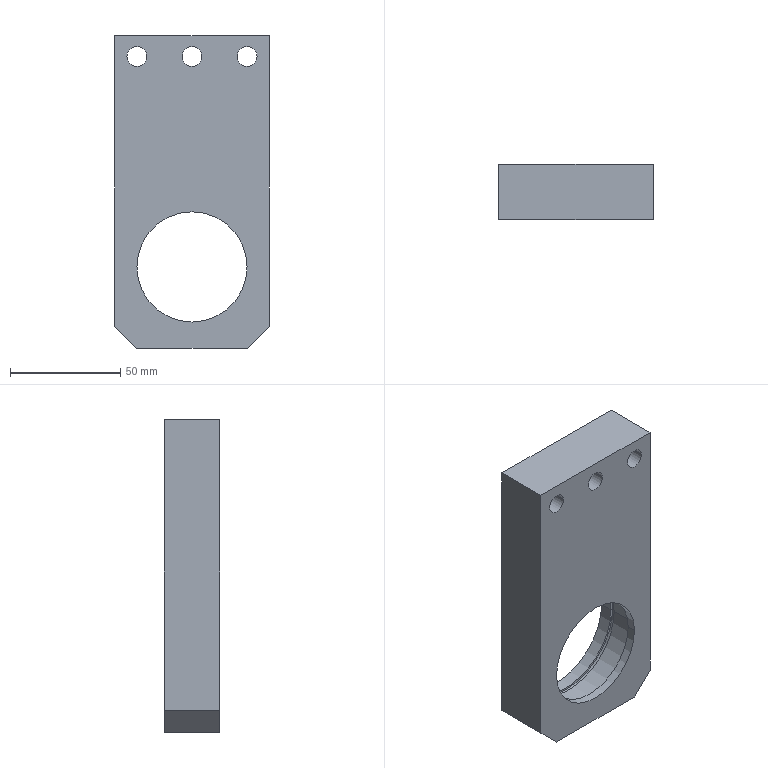Component | SolidWorks | -SlidingBearingHousing-1 | 1 solid | 34 faces | box 70 x 25 x 142 mm | volume 175353 mm3 | cylinder 20 | plane 14 | commonest cylinder face diameters 14 x6 9 x6 58 x4 60 x2 50 x2
build123d program:
from build123d import *

# Parameters (mm, degrees)
BOSS_EXTRUDE1_DEPTH = 25
SKETCH9_R           = 4.5
CUT_EXTRUDE5_DEPTH  = 84.012
SKETCH11_R          = 7
CUT_EXTRUDE6_DEPTH  = 8


with BuildPart() as part:
    # Sketch1 → Boss-Extrude1 (new body)
    with BuildSketch(Plane.XY):
        Polygon((-35, 61), (-25, 71), (25, 71), (35, 61), (35, -71), (-35, -71), align=None)
    extrude(amount=BOSS_EXTRUDE1_DEPTH)

    # Sketch9 → Cut-Extrude5 (cut, through all)
    with BuildSketch(Plane(origin=(0, 0, 0), x_dir=(-1, 0, 0), z_dir=(0, 0, -1))):
        with Locations((-25, -61.5)):
            Circle(SKETCH9_R)
        with Locations((0, -61.5)):
            Circle(SKETCH9_R)
        with Locations((25, -61.5)):
            Circle(SKETCH9_R)
    extrude(amount=-CUT_EXTRUDE5_DEPTH, mode=Mode.SUBTRACT)

    # Sketch10 → Cut-Revolve1 (revolve, cut)
    with BuildSketch(Plane(origin=(0, 0, 0), x_dir=(0, 0, -1), z_dir=(1, 0, 0)), mode=Mode.PRIVATE) as cut_revolve1_sk:
        Polygon((-25, 59), (-21, 59), (-21, 63), (-8, 63), (-8, 64), (-6, 64), (-6, 63), (0, 63), (0, 34), (-25, 34), align=None)
    revolve(cut_revolve1_sk.sketch.rotate(Axis((0, 34, 57.258), (0, 0, -1)), 90), axis=Axis((0, 34, 57.258), (0, 0, -1)), mode=Mode.SUBTRACT)

    # Sketch11 → Cut-Extrude6 (cut)
    with BuildSketch(Plane(origin=(0, 0, 0), x_dir=(-1, 0, 0), z_dir=(0, 0, -1))):
        with Locations((0, -61.5)):
            Circle(SKETCH11_R)
        with Locations((-25, -61.5)):
            Circle(SKETCH11_R)
        with Locations((25, -61.5)):
            Circle(SKETCH11_R)
    extrude(amount=-CUT_EXTRUDE6_DEPTH, mode=Mode.SUBTRACT)


solid = part.part

# Placed as in the assembly
solid = solid.moved(Location((205, 1334.5, -139), (90, 0, -180)))
STEP:
#1=COLOUR_RGB('',0.7922,0.8196,0.9333);
#2=FILL_AREA_STYLE_COLOUR('',#1);
#3=FILL_AREA_STYLE('',(#2));
#4=SURFACE_STYLE_FILL_AREA(#3);
#5=SURFACE_SIDE_STYLE('',(#4));
#6=SURFACE_STYLE_USAGE(.BOTH.,#5);
#7=PRESENTATION_STYLE_ASSIGNMENT((#6));
#8=CARTESIAN_POINT('',(8.78,52.224,-3.051));
#9=VERTEX_POINT('',#8);
#10=CARTESIAN_POINT('',(9.331,52.224,-3.051));
#11=VERTEX_POINT('',#10);
#12=CARTESIAN_POINT('',(9.055,52.224,-3.051));
#13=DIRECTION('',(-0.,1.,-0.));
#14=DIRECTION('',(1.,0.,0.));
#15=AXIS2_PLACEMENT_3D('',#12,#13,#14);
#16=CIRCLE('',#15,0.2756);
#17=EDGE_CURVE('',#9,#11,#16,.T.);
#18=ORIENTED_EDGE('',*,*,#17,.F.);
#19=CARTESIAN_POINT('',(8.78,52.539,-3.051));
#20=VERTEX_POINT('',#19);
#21=CARTESIAN_POINT('',(8.78,52.224,-3.051));
#22=DIRECTION('',(-0.,1.,-0.));
#23=VECTOR('',#22,39.37);
#24=LINE('',#21,#23);
#25=EDGE_CURVE('',#9,#20,#24,.T.);
#26=ORIENTED_EDGE('',*,*,#25,.T.);
#27=CARTESIAN_POINT('',(9.331,52.539,-3.051));
#28=VERTEX_POINT('',#27);
#29=CARTESIAN_POINT('',(9.055,52.539,-3.051));
#30=DIRECTION('',(-0.,1.,-0.));
#31=DIRECTION('',(1.,0.,0.));
#32=AXIS2_PLACEMENT_3D('',#29,#30,#31);
#33=CIRCLE('',#32,0.2756);
#34=EDGE_CURVE('',#20,#28,#33,.T.);
#35=ORIENTED_EDGE('',*,*,#34,.T.);
#36=CARTESIAN_POINT('',(9.331,52.224,-3.051));
#37=DIRECTION('',(-0.,1.,-0.));
#38=VECTOR('',#37,39.37);
#39=LINE('',#36,#38);
#40=EDGE_CURVE('',#11,#28,#39,.T.);
#41=ORIENTED_EDGE('',*,*,#40,.F.);
#42=EDGE_LOOP('',(#18,#26,#35,#41));
#43=FACE_OUTER_BOUND('',#42,.T.);
#44=CARTESIAN_POINT('',(9.055,52.224,-3.051));
#45=DIRECTION('',(-0.,1.,-0.));
#46=DIRECTION('',(1.,0.,0.));
#47=AXIS2_PLACEMENT_3D('',#44,#45,#46);
#48=CYLINDRICAL_SURFACE('',#47,0.2756);
#49=ADVANCED_FACE('',(#43),#48,.F.);
#50=CARTESIAN_POINT('',(6.811,52.224,-3.051));
#51=VERTEX_POINT('',#50);
#52=CARTESIAN_POINT('',(7.362,52.224,-3.051));
#53=VERTEX_POINT('',#52);
#54=CARTESIAN_POINT('',(7.087,52.224,-3.051));
#55=DIRECTION('',(-0.,1.,-0.));
#56=DIRECTION('',(1.,0.,0.));
#57=AXIS2_PLACEMENT_3D('',#54,#55,#56);
#58=CIRCLE('',#57,0.2756);
#59=EDGE_CURVE('',#51,#53,#58,.T.);
#60=ORIENTED_EDGE('',*,*,#59,.F.);
#61=CARTESIAN_POINT('',(6.811,52.539,-3.051));
#62=VERTEX_POINT('',#61);
#63=CARTESIAN_POINT('',(6.811,52.224,-3.051));
#64=DIRECTION('',(-0.,1.,-0.));
#65=VECTOR('',#64,39.37);
#66=LINE('',#63,#65);
#67=EDGE_CURVE('',#51,#62,#66,.T.);
#68=ORIENTED_EDGE('',*,*,#67,.T.);
#69=CARTESIAN_POINT('',(7.362,52.539,-3.051));
#70=VERTEX_POINT('',#69);
#71=CARTESIAN_POINT('',(7.087,52.539,-3.051));
#72=DIRECTION('',(-0.,1.,-0.));
#73=DIRECTION('',(1.,0.,0.));
#74=AXIS2_PLACEMENT_3D('',#71,#72,#73);
#75=CIRCLE('',#74,0.2756);
#76=EDGE_CURVE('',#62,#70,#75,.T.);
#77=ORIENTED_EDGE('',*,*,#76,.T.);
#78=CARTESIAN_POINT('',(7.362,52.224,-3.051));
#79=DIRECTION('',(-0.,1.,-0.));
#80=VECTOR('',#79,39.37);
#81=LINE('',#78,#80);
#82=EDGE_CURVE('',#53,#70,#81,.T.);
#83=ORIENTED_EDGE('',*,*,#82,.F.);
#84=EDGE_LOOP('',(#60,#68,#77,#83));
#85=FACE_OUTER_BOUND('',#84,.T.);
#86=CARTESIAN_POINT('',(7.087,52.224,-3.051));
#87=DIRECTION('',(-0.,1.,-0.));
#88=DIRECTION('',(1.,0.,0.));
#89=AXIS2_PLACEMENT_3D('',#86,#87,#88);
#90=CYLINDRICAL_SURFACE('',#89,0.2756);
#91=ADVANCED_FACE('',(#85),#90,.F.);
#92=CARTESIAN_POINT('',(7.795,52.224,-3.051));
#93=VERTEX_POINT('',#92);
#94=CARTESIAN_POINT('',(8.346,52.224,-3.051));
#95=VERTEX_POINT('',#94);
#96=CARTESIAN_POINT('',(8.071,52.224,-3.051));
#97=DIRECTION('',(-0.,1.,-0.));
#98=DIRECTION('',(1.,0.,0.));
#99=AXIS2_PLACEMENT_3D('',#96,#97,#98);
#100=CIRCLE('',#99,0.2756);
#101=EDGE_CURVE('',#93,#95,#100,.T.);
#102=ORIENTED_EDGE('',*,*,#101,.F.);
#103=CARTESIAN_POINT('',(7.795,52.539,-3.051));
#104=VERTEX_POINT('',#103);
#105=CARTESIAN_POINT('',(7.795,52.224,-3.051));
#106=DIRECTION('',(-0.,1.,-0.));
#107=VECTOR('',#106,39.37);
#108=LINE('',#105,#107);
#109=EDGE_CURVE('',#93,#104,#108,.T.);
#110=ORIENTED_EDGE('',*,*,#109,.T.);
#111=CARTESIAN_POINT('',(8.346,52.539,-3.051));
#112=VERTEX_POINT('',#111);
#113=CARTESIAN_POINT('',(8.071,52.539,-3.051));
#114=DIRECTION('',(-0.,1.,-0.));
#115=DIRECTION('',(1.,0.,0.));
#116=AXIS2_PLACEMENT_3D('',#113,#114,#115);
#117=CIRCLE('',#116,0.2756);
#118=EDGE_CURVE('',#104,#112,#117,.T.);
#119=ORIENTED_EDGE('',*,*,#118,.T.);
#120=CARTESIAN_POINT('',(8.346,52.224,-3.051));
#121=DIRECTION('',(-0.,1.,-0.));
#122=VECTOR('',#121,39.37);
#123=LINE('',#120,#122);
#124=EDGE_CURVE('',#95,#112,#123,.T.);
#125=ORIENTED_EDGE('',*,*,#124,.F.);
#126=EDGE_LOOP('',(#102,#110,#119,#125));
#127=FACE_OUTER_BOUND('',#126,.T.);
#128=CARTESIAN_POINT('',(8.071,52.224,-3.051));
#129=DIRECTION('',(-0.,1.,-0.));
#130=DIRECTION('',(1.,0.,0.));
#131=AXIS2_PLACEMENT_3D('',#128,#129,#130);
#132=CYLINDRICAL_SURFACE('',#131,0.2756);
#133=ADVANCED_FACE('',(#127),#132,.F.);
#134=CARTESIAN_POINT('',(9.213,52.539,-6.811));
#135=VERTEX_POINT('',#134);
#136=CARTESIAN_POINT('',(6.929,52.539,-6.811));
#137=VERTEX_POINT('',#136);
#138=CARTESIAN_POINT('',(8.071,52.539,-6.811));
#139=DIRECTION('',(0.,-1.,0.));
#140=DIRECTION('',(-1.,0.,0.));
#141=AXIS2_PLACEMENT_3D('',#138,#139,#140);
#142=CIRCLE('',#141,1.142);
#143=EDGE_CURVE('',#135,#137,#142,.T.);
#144=ORIENTED_EDGE('',*,*,#143,.F.);
#145=CARTESIAN_POINT('',(9.213,52.303,-6.811));
#146=VERTEX_POINT('',#145);
#147=CARTESIAN_POINT('',(9.213,50.285,-6.811));
#148=DIRECTION('',(0.,-1.,0.));
#149=VECTOR('',#148,39.37);
#150=LINE('',#147,#149);
#151=EDGE_CURVE('',#135,#146,#150,.T.);
#152=ORIENTED_EDGE('',*,*,#151,.T.);
#153=CARTESIAN_POINT('',(6.929,52.303,-6.811));
#154=VERTEX_POINT('',#153);
#155=CARTESIAN_POINT('',(8.071,52.303,-6.811));
#156=DIRECTION('',(0.,-1.,0.));
#157=DIRECTION('',(-1.,0.,0.));
#158=AXIS2_PLACEMENT_3D('',#155,#156,#157);
#159=CIRCLE('',#158,1.142);
#160=EDGE_CURVE('',#146,#154,#159,.T.);
#161=ORIENTED_EDGE('',*,*,#160,.T.);
#162=CARTESIAN_POINT('',(6.929,50.285,-6.811));
#163=DIRECTION('',(0.,-1.,0.));
#164=VECTOR('',#163,39.37);
#165=LINE('',#162,#164);
#166=EDGE_CURVE('',#137,#154,#165,.T.);
#167=ORIENTED_EDGE('',*,*,#166,.F.);
#168=EDGE_LOOP('',(#144,#152,#161,#167));
#169=FACE_OUTER_BOUND('',#168,.T.);
#170=CARTESIAN_POINT('',(8.071,50.285,-6.811));
#171=DIRECTION('',(0.,-1.,0.));
#172=DIRECTION('',(-1.,0.,0.));
#173=AXIS2_PLACEMENT_3D('',#170,#171,#172);
#174=CYLINDRICAL_SURFACE('',#173,1.142);
#175=ADVANCED_FACE('',(#169),#174,.F.);
#176=CARTESIAN_POINT('',(9.252,52.303,-6.811));
#177=VERTEX_POINT('',#176);
#178=CARTESIAN_POINT('',(6.89,52.303,-6.811));
#179=VERTEX_POINT('',#178);
#180=CARTESIAN_POINT('',(8.071,52.303,-6.811));
#181=DIRECTION('',(0.,-1.,0.));
#182=DIRECTION('',(-1.,0.,0.));
#183=AXIS2_PLACEMENT_3D('',#180,#181,#182);
#184=CIRCLE('',#183,1.181);
#185=EDGE_CURVE('',#177,#179,#184,.T.);
#186=ORIENTED_EDGE('',*,*,#185,.F.);
#187=CARTESIAN_POINT('',(9.252,52.224,-6.811));
#188=VERTEX_POINT('',#187);
#189=CARTESIAN_POINT('',(9.252,50.285,-6.811));
#190=DIRECTION('',(0.,-1.,0.));
#191=VECTOR('',#190,39.37);
#192=LINE('',#189,#191);
#193=EDGE_CURVE('',#177,#188,#192,.T.);
#194=ORIENTED_EDGE('',*,*,#193,.T.);
#195=CARTESIAN_POINT('',(6.89,52.224,-6.811));
#196=VERTEX_POINT('',#195);
#197=CARTESIAN_POINT('',(8.071,52.224,-6.811));
#198=DIRECTION('',(0.,-1.,0.));
#199=DIRECTION('',(-1.,0.,0.));
#200=AXIS2_PLACEMENT_3D('',#197,#198,#199);
#201=CIRCLE('',#200,1.181);
#202=EDGE_CURVE('',#188,#196,#201,.T.);
#203=ORIENTED_EDGE('',*,*,#202,.T.);
#204=CARTESIAN_POINT('',(6.89,50.285,-6.811));
#205=DIRECTION('',(0.,-1.,0.));
#206=VECTOR('',#205,39.37);
#207=LINE('',#204,#206);
#208=EDGE_CURVE('',#179,#196,#207,.T.);
#209=ORIENTED_EDGE('',*,*,#208,.F.);
#210=EDGE_LOOP('',(#186,#194,#203,#209));
#211=FACE_OUTER_BOUND('',#210,.T.);
#212=CARTESIAN_POINT('',(8.071,50.285,-6.811));
#213=DIRECTION('',(0.,-1.,0.));
#214=DIRECTION('',(-1.,0.,0.));
#215=AXIS2_PLACEMENT_3D('',#212,#213,#214);
#216=CYLINDRICAL_SURFACE('',#215,1.181);
#217=ADVANCED_FACE('',(#211),#216,.F.);
#218=CARTESIAN_POINT('',(9.213,52.224,-6.811));
#219=VERTEX_POINT('',#218);
#220=CARTESIAN_POINT('',(6.929,52.224,-6.811));
#221=VERTEX_POINT('',#220);
#222=CARTESIAN_POINT('',(8.071,52.224,-6.811));
#223=DIRECTION('',(0.,-1.,0.));
#224=DIRECTION('',(-1.,0.,0.));
#225=AXIS2_PLACEMENT_3D('',#222,#223,#224);
#226=CIRCLE('',#225,1.142);
#227=EDGE_CURVE('',#219,#221,#226,.T.);
#228=ORIENTED_EDGE('',*,*,#227,.F.);
#229=CARTESIAN_POINT('',(9.213,51.713,-6.811));
#230=VERTEX_POINT('',#229);
#231=CARTESIAN_POINT('',(9.213,50.285,-6.811));
#232=DIRECTION('',(0.,-1.,0.));
#233=VECTOR('',#232,39.37);
#234=LINE('',#231,#233);
#235=EDGE_CURVE('',#219,#230,#234,.T.);
#236=ORIENTED_EDGE('',*,*,#235,.T.);
#237=CARTESIAN_POINT('',(6.929,51.713,-6.811));
#238=VERTEX_POINT('',#237);
#239=CARTESIAN_POINT('',(8.071,51.713,-6.811));
#240=DIRECTION('',(0.,-1.,0.));
#241=DIRECTION('',(-1.,0.,0.));
#242=AXIS2_PLACEMENT_3D('',#239,#240,#241);
#243=CIRCLE('',#242,1.142);
#244=EDGE_CURVE('',#230,#238,#243,.T.);
#245=ORIENTED_EDGE('',*,*,#244,.T.);
#246=CARTESIAN_POINT('',(6.929,50.285,-6.811));
#247=DIRECTION('',(0.,-1.,0.));
#248=VECTOR('',#247,39.37);
#249=LINE('',#246,#248);
#250=EDGE_CURVE('',#221,#238,#249,.T.);
#251=ORIENTED_EDGE('',*,*,#250,.F.);
#252=EDGE_LOOP('',(#228,#236,#245,#251));
#253=FACE_OUTER_BOUND('',#252,.T.);
#254=CARTESIAN_POINT('',(8.071,50.285,-6.811));
#255=DIRECTION('',(0.,-1.,0.));
#256=DIRECTION('',(-1.,0.,0.));
#257=AXIS2_PLACEMENT_3D('',#254,#255,#256);
#258=CYLINDRICAL_SURFACE('',#257,1.142);
#259=ADVANCED_FACE('',(#253),#258,.F.);
#260=CARTESIAN_POINT('',(9.055,51.713,-6.811));
#261=VERTEX_POINT('',#260);
#262=CARTESIAN_POINT('',(7.087,51.713,-6.811));
#263=VERTEX_POINT('',#262);
#264=CARTESIAN_POINT('',(8.071,51.713,-6.811));
#265=DIRECTION('',(0.,-1.,0.));
#266=DIRECTION('',(-1.,0.,0.));
#267=AXIS2_PLACEMENT_3D('',#264,#265,#266);
#268=CIRCLE('',#267,0.9843);
#269=EDGE_CURVE('',#261,#263,#268,.T.);
#270=ORIENTED_EDGE('',*,*,#269,.F.);
#271=CARTESIAN_POINT('',(9.055,51.555,-6.811));
#272=VERTEX_POINT('',#271);
#273=CARTESIAN_POINT('',(9.055,50.285,-6.811));
#274=DIRECTION('',(0.,-1.,0.));
#275=VECTOR('',#274,39.37);
#276=LINE('',#273,#275);
#277=EDGE_CURVE('',#261,#272,#276,.T.);
#278=ORIENTED_EDGE('',*,*,#277,.T.);
#279=CARTESIAN_POINT('',(7.087,51.555,-6.811));
#280=VERTEX_POINT('',#279);
#281=CARTESIAN_POINT('',(8.071,51.555,-6.811));
#282=DIRECTION('',(0.,-1.,0.));
#283=DIRECTION('',(-1.,0.,0.));
#284=AXIS2_PLACEMENT_3D('',#281,#282,#283);
#285=CIRCLE('',#284,0.9843);
#286=EDGE_CURVE('',#272,#280,#285,.T.);
#287=ORIENTED_EDGE('',*,*,#286,.T.);
#288=CARTESIAN_POINT('',(7.087,50.285,-6.811));
#289=DIRECTION('',(0.,-1.,0.));
#290=VECTOR('',#289,39.37);
#291=LINE('',#288,#290);
#292=EDGE_CURVE('',#263,#280,#291,.T.);
#293=ORIENTED_EDGE('',*,*,#292,.F.);
#294=EDGE_LOOP('',(#270,#278,#287,#293));
#295=FACE_OUTER_BOUND('',#294,.T.);
#296=CARTESIAN_POINT('',(8.071,50.285,-6.811));
#297=DIRECTION('',(0.,-1.,0.));
#298=DIRECTION('',(-1.,0.,0.));
#299=AXIS2_PLACEMENT_3D('',#296,#297,#298);
#300=CYLINDRICAL_SURFACE('',#299,0.9843);
#301=ADVANCED_FACE('',(#295),#300,.F.);
#302=CARTESIAN_POINT('',(7.894,51.555,-3.051));
#303=VERTEX_POINT('',#302);
#304=CARTESIAN_POINT('',(8.248,51.555,-3.051));
#305=VERTEX_POINT('',#304);
#306=CARTESIAN_POINT('',(8.071,51.555,-3.051));
#307=DIRECTION('',(-0.,1.,-0.));
#308=DIRECTION('',(1.,0.,0.));
#309=AXIS2_PLACEMENT_3D('',#306,#307,#308);
#310=CIRCLE('',#309,0.1772);
#311=EDGE_CURVE('',#303,#305,#310,.T.);
#312=ORIENTED_EDGE('',*,*,#311,.F.);
#313=CARTESIAN_POINT('',(7.894,52.224,-3.051));
#314=VERTEX_POINT('',#313);
#315=CARTESIAN_POINT('',(7.894,51.555,-3.051));
#316=DIRECTION('',(-0.,1.,-0.));
#317=VECTOR('',#316,39.37);
#318=LINE('',#315,#317);
#319=EDGE_CURVE('',#303,#314,#318,.T.);
#320=ORIENTED_EDGE('',*,*,#319,.T.);
#321=CARTESIAN_POINT('',(8.248,52.224,-3.051));
#322=VERTEX_POINT('',#321);
#323=CARTESIAN_POINT('',(8.071,52.224,-3.051));
#324=DIRECTION('',(0.,-1.,0.));
#325=DIRECTION('',(1.,0.,0.));
#326=AXIS2_PLACEMENT_3D('',#323,#324,#325);
#327=CIRCLE('',#326,0.1772);
#328=EDGE_CURVE('',#322,#314,#327,.T.);
#329=ORIENTED_EDGE('',*,*,#328,.F.);
#330=CARTESIAN_POINT('',(8.248,51.555,-3.051));
#331=DIRECTION('',(-0.,1.,-0.));
#332=VECTOR('',#331,39.37);
#333=LINE('',#330,#332);
#334=EDGE_CURVE('',#305,#322,#333,.T.);
#335=ORIENTED_EDGE('',*,*,#334,.F.);
#336=EDGE_LOOP('',(#312,#320,#329,#335));
#337=FACE_OUTER_BOUND('',#336,.T.);
#338=CARTESIAN_POINT('',(8.071,51.555,-3.051));
#339=DIRECTION('',(-0.,1.,-0.));
#340=DIRECTION('',(1.,0.,0.));
#341=AXIS2_PLACEMENT_3D('',#338,#339,#340);
#342=CYLINDRICAL_SURFACE('',#341,0.1772);
#343=ADVANCED_FACE('',(#337),#342,.F.);
#344=CARTESIAN_POINT('',(6.909,51.555,-3.051));
#345=VERTEX_POINT('',#344);
#346=CARTESIAN_POINT('',(7.264,51.555,-3.051));
#347=VERTEX_POINT('',#346);
#348=CARTESIAN_POINT('',(7.087,51.555,-3.051));
#349=DIRECTION('',(-0.,1.,-0.));
#350=DIRECTION('',(1.,0.,0.));
#351=AXIS2_PLACEMENT_3D('',#348,#349,#350);
#352=CIRCLE('',#351,0.1772);
#353=EDGE_CURVE('',#345,#347,#352,.T.);
#354=ORIENTED_EDGE('',*,*,#353,.F.);
#355=CARTESIAN_POINT('',(6.909,52.224,-3.051));
#356=VERTEX_POINT('',#355);
#357=CARTESIAN_POINT('',(6.909,51.555,-3.051));
#358=DIRECTION('',(-0.,1.,-0.));
#359=VECTOR('',#358,39.37);
#360=LINE('',#357,#359);
#361=EDGE_CURVE('',#345,#356,#360,.T.);
#362=ORIENTED_EDGE('',*,*,#361,.T.);
#363=CARTESIAN_POINT('',(7.264,52.224,-3.051));
#364=VERTEX_POINT('',#363);
#365=CARTESIAN_POINT('',(7.087,52.224,-3.051));
#366=DIRECTION('',(0.,-1.,0.));
#367=DIRECTION('',(1.,0.,0.));
#368=AXIS2_PLACEMENT_3D('',#365,#366,#367);
#369=CIRCLE('',#368,0.1772);
#370=EDGE_CURVE('',#364,#356,#369,.T.);
#371=ORIENTED_EDGE('',*,*,#370,.F.);
#372=CARTESIAN_POINT('',(7.264,51.555,-3.051));
#373=DIRECTION('',(-0.,1.,-0.));
#374=VECTOR('',#373,39.37);
#375=LINE('',#372,#374);
#376=EDGE_CURVE('',#347,#364,#375,.T.);
#377=ORIENTED_EDGE('',*,*,#376,.F.);
#378=EDGE_LOOP('',(#354,#362,#371,#377));
#379=FACE_OUTER_BOUND('',#378,.T.);
#380=CARTESIAN_POINT('',(7.087,51.555,-3.051));
#381=DIRECTION('',(-0.,1.,-0.));
#382=DIRECTION('',(1.,0.,0.));
#383=AXIS2_PLACEMENT_3D('',#380,#381,#382);
#384=CYLINDRICAL_SURFACE('',#383,0.1772);
#385=ADVANCED_FACE('',(#379),#384,.F.);
#386=CARTESIAN_POINT('',(8.878,51.555,-3.051));
#387=VERTEX_POINT('',#386);
#388=CARTESIAN_POINT('',(9.232,51.555,-3.051));
#389=VERTEX_POINT('',#388);
#390=CARTESIAN_POINT('',(9.055,51.555,-3.051));
#391=DIRECTION('',(-0.,1.,-0.));
#392=DIRECTION('',(1.,0.,0.));
#393=AXIS2_PLACEMENT_3D('',#390,#391,#392);
#394=CIRCLE('',#393,0.1772);
#395=EDGE_CURVE('',#387,#389,#394,.T.);
#396=ORIENTED_EDGE('',*,*,#395,.F.);
#397=CARTESIAN_POINT('',(8.878,52.224,-3.051));
#398=VERTEX_POINT('',#397);
#399=CARTESIAN_POINT('',(8.878,51.555,-3.051));
#400=DIRECTION('',(-0.,1.,-0.));
#401=VECTOR('',#400,39.37);
#402=LINE('',#399,#401);
#403=EDGE_CURVE('',#387,#398,#402,.T.);
#404=ORIENTED_EDGE('',*,*,#403,.T.);
#405=CARTESIAN_POINT('',(9.232,52.224,-3.051));
#406=VERTEX_POINT('',#405);
#407=CARTESIAN_POINT('',(9.055,52.224,-3.051));
#408=DIRECTION('',(0.,-1.,0.));
#409=DIRECTION('',(1.,0.,0.));
#410=AXIS2_PLACEMENT_3D('',#407,#408,#409);
#411=CIRCLE('',#410,0.1772);
#412=EDGE_CURVE('',#406,#398,#411,.T.);
#413=ORIENTED_EDGE('',*,*,#412,.F.);
#414=CARTESIAN_POINT('',(9.232,51.555,-3.051));
#415=DIRECTION('',(-0.,1.,-0.));
#416=VECTOR('',#415,39.37);
#417=LINE('',#414,#416);
#418=EDGE_CURVE('',#389,#406,#417,.T.);
#419=ORIENTED_EDGE('',*,*,#418,.F.);
#420=EDGE_LOOP('',(#396,#404,#413,#419));
#421=FACE_OUTER_BOUND('',#420,.T.);
#422=CARTESIAN_POINT('',(9.055,51.555,-3.051));
#423=DIRECTION('',(-0.,1.,-0.));
#424=DIRECTION('',(1.,0.,0.));
#425=AXIS2_PLACEMENT_3D('',#422,#423,#424);
#426=CYLINDRICAL_SURFACE('',#425,0.1772);
#427=ADVANCED_FACE('',(#421),#426,.F.);
#428=ORIENTED_EDGE('',*,*,#403,.F.);
#429=CARTESIAN_POINT('',(9.055,51.555,-3.051));
#430=DIRECTION('',(-0.,1.,-0.));
#431=DIRECTION('',(1.,0.,0.));
#432=AXIS2_PLACEMENT_3D('',#429,#430,#431);
#433=CIRCLE('',#432,0.1772);
#434=EDGE_CURVE('',#389,#387,#433,.T.);
#435=ORIENTED_EDGE('',*,*,#434,.F.);
#436=ORIENTED_EDGE('',*,*,#418,.T.);
#437=CARTESIAN_POINT('',(9.055,52.224,-3.051));
#438=DIRECTION('',(0.,-1.,0.));
#439=DIRECTION('',(1.,0.,0.));
#440=AXIS2_PLACEMENT_3D('',#437,#438,#439);
#441=CIRCLE('',#440,0.1772);
#442=EDGE_CURVE('',#398,#406,#441,.T.);
#443=ORIENTED_EDGE('',*,*,#442,.F.);
#444=EDGE_LOOP('',(#428,#435,#436,#443));
#445=FACE_OUTER_BOUND('',#444,.T.);
#446=CARTESIAN_POINT('',(9.055,51.555,-3.051));
#447=DIRECTION('',(-0.,1.,-0.));
#448=DIRECTION('',(1.,0.,0.));
#449=AXIS2_PLACEMENT_3D('',#446,#447,#448);
#450=CYLINDRICAL_SURFACE('',#449,0.1772);
#451=ADVANCED_FACE('',(#445),#450,.F.);
#452=ORIENTED_EDGE('',*,*,#361,.F.);
#453=CARTESIAN_POINT('',(7.087,51.555,-3.051));
#454=DIRECTION('',(-0.,1.,-0.));
#455=DIRECTION('',(1.,0.,0.));
#456=AXIS2_PLACEMENT_3D('',#453,#454,#455);
#457=CIRCLE('',#456,0.1772);
#458=EDGE_CURVE('',#347,#345,#457,.T.);
#459=ORIENTED_EDGE('',*,*,#458,.F.);
#460=ORIENTED_EDGE('',*,*,#376,.T.);
#461=CARTESIAN_POINT('',(7.087,52.224,-3.051));
#462=DIRECTION('',(0.,-1.,0.));
#463=DIRECTION('',(1.,0.,0.));
#464=AXIS2_PLACEMENT_3D('',#461,#462,#463);
#465=CIRCLE('',#464,0.1772);
#466=EDGE_CURVE('',#356,#364,#465,.T.);
#467=ORIENTED_EDGE('',*,*,#466,.F.);
#468=EDGE_LOOP('',(#452,#459,#460,#467));
#469=FACE_OUTER_BOUND('',#468,.T.);
#470=CARTESIAN_POINT('',(7.087,51.555,-3.051));
#471=DIRECTION('',(-0.,1.,-0.));
#472=DIRECTION('',(1.,0.,0.));
#473=AXIS2_PLACEMENT_3D('',#470,#471,#472);
#474=CYLINDRICAL_SURFACE('',#473,0.1772);
#475=ADVANCED_FACE('',(#469),#474,.F.);
#476=ORIENTED_EDGE('',*,*,#319,.F.);
#477=CARTESIAN_POINT('',(8.071,51.555,-3.051));
#478=DIRECTION('',(-0.,1.,-0.));
#479=DIRECTION('',(1.,0.,0.));
#480=AXIS2_PLACEMENT_3D('',#477,#478,#479);
#481=CIRCLE('',#480,0.1772);
#482=EDGE_CURVE('',#305,#303,#481,.T.);
#483=ORIENTED_EDGE('',*,*,#482,.F.);
#484=ORIENTED_EDGE('',*,*,#334,.T.);
#485=CARTESIAN_POINT('',(8.071,52.224,-3.051));
#486=DIRECTION('',(0.,-1.,0.));
#487=DIRECTION('',(1.,0.,0.));
#488=AXIS2_PLACEMENT_3D('',#485,#486,#487);
#489=CIRCLE('',#488,0.1772);
#490=EDGE_CURVE('',#314,#322,#489,.T.);
#491=ORIENTED_EDGE('',*,*,#490,.F.);
#492=EDGE_LOOP('',(#476,#483,#484,#491));
#493=FACE_OUTER_BOUND('',#492,.T.);
#494=CARTESIAN_POINT('',(8.071,51.555,-3.051));
#495=DIRECTION('',(-0.,1.,-0.));
#496=DIRECTION('',(1.,0.,0.));
#497=AXIS2_PLACEMENT_3D('',#494,#495,#496);
#498=CYLINDRICAL_SURFACE('',#497,0.1772);
#499=ADVANCED_FACE('',(#493),#498,.F.);
#500=CARTESIAN_POINT('',(6.693,51.555,-2.677));
#501=VERTEX_POINT('',#500);
#502=CARTESIAN_POINT('',(6.693,51.555,-7.874));
#503=VERTEX_POINT('',#502);
#504=CARTESIAN_POINT('',(6.693,51.555,-7.874));
#505=DIRECTION('',(-0.,-0.,-1.));
#506=VECTOR('',#505,39.37);
#507=LINE('',#504,#506);
#508=EDGE_CURVE('',#501,#503,#507,.T.);
#509=ORIENTED_EDGE('',*,*,#508,.T.);
#510=CARTESIAN_POINT('',(7.087,51.555,-8.268));
#511=VERTEX_POINT('',#510);
#512=CARTESIAN_POINT('',(7.087,51.555,-8.268));
#513=DIRECTION('',(0.7071,-0.,-0.7071));
#514=VECTOR('',#513,39.37);
#515=LINE('',#512,#514);
#516=EDGE_CURVE('',#503,#511,#515,.T.);
#517=ORIENTED_EDGE('',*,*,#516,.T.);
#518=CARTESIAN_POINT('',(9.055,51.555,-8.268));
#519=VERTEX_POINT('',#518);
#520=CARTESIAN_POINT('',(9.055,51.555,-8.268));
#521=DIRECTION('',(1.,0.,-0.));
#522=VECTOR('',#521,39.37);
#523=LINE('',#520,#522);
#524=EDGE_CURVE('',#511,#519,#523,.T.);
#525=ORIENTED_EDGE('',*,*,#524,.T.);
#526=CARTESIAN_POINT('',(9.449,51.555,-7.874));
#527=VERTEX_POINT('',#526);
#528=CARTESIAN_POINT('',(9.449,51.555,-7.874));
#529=DIRECTION('',(0.7071,0.,0.7071));
#530=VECTOR('',#529,39.37);
#531=LINE('',#528,#530);
#532=EDGE_CURVE('',#519,#527,#531,.T.);
#533=ORIENTED_EDGE('',*,*,#532,.T.);
#534=CARTESIAN_POINT('',(9.449,51.555,-2.677));
#535=VERTEX_POINT('',#534);
#536=CARTESIAN_POINT('',(9.449,51.555,-7.874));
#537=DIRECTION('',(0.,0.,1.));
#538=VECTOR('',#537,39.37);
#539=LINE('',#536,#538);
#540=EDGE_CURVE('',#527,#535,#539,.T.);
#541=ORIENTED_EDGE('',*,*,#540,.T.);
#542=CARTESIAN_POINT('',(9.449,51.555,-2.677));
#543=DIRECTION('',(-1.,-0.,0.));
#544=VECTOR('',#543,39.37);
#545=LINE('',#542,#544);
#546=EDGE_CURVE('',#535,#501,#545,.T.);
#547=ORIENTED_EDGE('',*,*,#546,.T.);
#548=EDGE_LOOP('',(#509,#517,#525,#533,#541,#547));
#549=FACE_OUTER_BOUND('',#548,.T.);
#550=ORIENTED_EDGE('',*,*,#458,.T.);
#551=ORIENTED_EDGE('',*,*,#353,.T.);
#552=EDGE_LOOP('',(#550,#551));
#553=FACE_BOUND('',#552,.T.);
#554=ORIENTED_EDGE('',*,*,#482,.T.);
#555=ORIENTED_EDGE('',*,*,#311,.T.);
#556=EDGE_LOOP('',(#554,#555));
#557=FACE_BOUND('',#556,.T.);
#558=ORIENTED_EDGE('',*,*,#434,.T.);
#559=ORIENTED_EDGE('',*,*,#395,.T.);
#560=EDGE_LOOP('',(#558,#559));
#561=FACE_BOUND('',#560,.T.);
#562=CARTESIAN_POINT('',(8.071,51.555,-6.811));
#563=DIRECTION('',(0.,-1.,0.));
#564=DIRECTION('',(-1.,0.,0.));
#565=AXIS2_PLACEMENT_3D('',#562,#563,#564);
#566=CIRCLE('',#565,0.9843);
#567=EDGE_CURVE('',#280,#272,#566,.T.);
#568=ORIENTED_EDGE('',*,*,#567,.F.);
#569=ORIENTED_EDGE('',*,*,#286,.F.);
#570=EDGE_LOOP('',(#568,#569));
#571=FACE_BOUND('',#570,.T.);
#572=CARTESIAN_POINT('',(8.071,51.555,-5.472));
#573=DIRECTION('',(0.,-1.,0.));
#574=DIRECTION('',(-1.,-0.,0.));
#575=AXIS2_PLACEMENT_3D('',#572,#573,#574);
#576=PLANE('',#575);
#577=ADVANCED_FACE('',(#549,#553,#557,#561,#571),#576,.T.);
#578=CARTESIAN_POINT('',(9.055,52.539,-3.051));
#579=DIRECTION('',(-0.,1.,-0.));
#580=DIRECTION('',(1.,0.,0.));
#581=AXIS2_PLACEMENT_3D('',#578,#579,#580);
#582=CIRCLE('',#581,0.2756);
#583=EDGE_CURVE('',#28,#20,#582,.T.);
#584=ORIENTED_EDGE('',*,*,#583,.F.);
#585=ORIENTED_EDGE('',*,*,#34,.F.);
#586=EDGE_LOOP('',(#584,#585));
#587=FACE_BOUND('',#586,.T.);
#588=CARTESIAN_POINT('',(7.087,52.539,-3.051));
#589=DIRECTION('',(-0.,1.,-0.));
#590=DIRECTION('',(1.,0.,0.));
#591=AXIS2_PLACEMENT_3D('',#588,#589,#590);
#592=CIRCLE('',#591,0.2756);
#593=EDGE_CURVE('',#70,#62,#592,.T.);
#594=ORIENTED_EDGE('',*,*,#593,.F.);
#595=ORIENTED_EDGE('',*,*,#76,.F.);
#596=EDGE_LOOP('',(#594,#595));
#597=FACE_BOUND('',#596,.T.);
#598=CARTESIAN_POINT('',(8.071,52.539,-3.051));
#599=DIRECTION('',(-0.,1.,-0.));
#600=DIRECTION('',(1.,0.,0.));
#601=AXIS2_PLACEMENT_3D('',#598,#599,#600);
#602=CIRCLE('',#601,0.2756);
#603=EDGE_CURVE('',#112,#104,#602,.T.);
#604=ORIENTED_EDGE('',*,*,#603,.F.);
#605=ORIENTED_EDGE('',*,*,#118,.F.);
#606=EDGE_LOOP('',(#604,#605));
#607=FACE_BOUND('',#606,.T.);
#608=CARTESIAN_POINT('',(6.693,52.539,-2.677));
#609=VERTEX_POINT('',#608);
#610=CARTESIAN_POINT('',(6.693,52.539,-7.874));
#611=VERTEX_POINT('',#610);
#612=CARTESIAN_POINT('',(6.693,52.539,-7.874));
#613=DIRECTION('',(-0.,-0.,-1.));
#614=VECTOR('',#613,39.37);
#615=LINE('',#612,#614);
#616=EDGE_CURVE('',#609,#611,#615,.T.);
#617=ORIENTED_EDGE('',*,*,#616,.F.);
#618=CARTESIAN_POINT('',(9.449,52.539,-2.677));
#619=VERTEX_POINT('',#618);
#620=CARTESIAN_POINT('',(9.449,52.539,-2.677));
#621=DIRECTION('',(-1.,-0.,0.));
#622=VECTOR('',#621,39.37);
#623=LINE('',#620,#622);
#624=EDGE_CURVE('',#619,#609,#623,.T.);
#625=ORIENTED_EDGE('',*,*,#624,.F.);
#626=CARTESIAN_POINT('',(9.449,52.539,-7.874));
#627=VERTEX_POINT('',#626);
#628=CARTESIAN_POINT('',(9.449,52.539,-7.874));
#629=DIRECTION('',(0.,0.,1.));
#630=VECTOR('',#629,39.37);
#631=LINE('',#628,#630);
#632=EDGE_CURVE('',#627,#619,#631,.T.);
#633=ORIENTED_EDGE('',*,*,#632,.F.);
#634=CARTESIAN_POINT('',(9.055,52.539,-8.268));
#635=VERTEX_POINT('',#634);
#636=CARTESIAN_POINT('',(9.449,52.539,-7.874));
#637=DIRECTION('',(0.7071,0.,0.7071));
#638=VECTOR('',#637,39.37);
#639=LINE('',#636,#638);
#640=EDGE_CURVE('',#635,#627,#639,.T.);
#641=ORIENTED_EDGE('',*,*,#640,.F.);
#642=CARTESIAN_POINT('',(7.087,52.539,-8.268));
#643=VERTEX_POINT('',#642);
#644=CARTESIAN_POINT('',(9.055,52.539,-8.268));
#645=DIRECTION('',(1.,0.,-0.));
#646=VECTOR('',#645,39.37);
#647=LINE('',#644,#646);
#648=EDGE_CURVE('',#643,#635,#647,.T.);
#649=ORIENTED_EDGE('',*,*,#648,.F.);
#650=CARTESIAN_POINT('',(7.087,52.539,-8.268));
#651=DIRECTION('',(0.7071,-0.,-0.7071));
#652=VECTOR('',#651,39.37);
#653=LINE('',#650,#652);
#654=EDGE_CURVE('',#611,#643,#653,.T.);
#655=ORIENTED_EDGE('',*,*,#654,.F.);
#656=EDGE_LOOP('',(#617,#625,#633,#641,#649,#655));
#657=FACE_OUTER_BOUND('',#656,.T.);
#658=CARTESIAN_POINT('',(8.071,52.539,-6.811));
#659=DIRECTION('',(0.,-1.,0.));
#660=DIRECTION('',(-1.,0.,0.));
#661=AXIS2_PLACEMENT_3D('',#658,#659,#660);
#662=CIRCLE('',#661,1.142);
#663=EDGE_CURVE('',#137,#135,#662,.T.);
#664=ORIENTED_EDGE('',*,*,#663,.T.);
#665=ORIENTED_EDGE('',*,*,#143,.T.);
#666=EDGE_LOOP('',(#664,#665));
#667=FACE_BOUND('',#666,.T.);
#668=CARTESIAN_POINT('',(8.071,52.539,-5.472));
#669=DIRECTION('',(0.,-1.,0.));
#670=DIRECTION('',(-1.,-0.,0.));
#671=AXIS2_PLACEMENT_3D('',#668,#669,#670);
#672=PLANE('',#671);
#673=ADVANCED_FACE('',(#587,#597,#607,#657,#667),#672,.F.);
#674=ORIENTED_EDGE('',*,*,#616,.T.);
#675=CARTESIAN_POINT('',(6.693,51.555,-7.874));
#676=DIRECTION('',(-0.,1.,-0.));
#677=VECTOR('',#676,39.37);
#678=LINE('',#675,#677);
#679=EDGE_CURVE('',#503,#611,#678,.T.);
#680=ORIENTED_EDGE('',*,*,#679,.F.);
#681=ORIENTED_EDGE('',*,*,#508,.F.);
#682=CARTESIAN_POINT('',(6.693,51.555,-2.677));
#683=DIRECTION('',(-0.,1.,-0.));
#684=VECTOR('',#683,39.37);
#685=LINE('',#682,#684);
#686=EDGE_CURVE('',#501,#609,#685,.T.);
#687=ORIENTED_EDGE('',*,*,#686,.T.);
#688=EDGE_LOOP('',(#674,#680,#681,#687));
#689=FACE_OUTER_BOUND('',#688,.T.);
#690=CARTESIAN_POINT('',(6.693,51.555,-7.874));
#691=DIRECTION('',(1.,0.,-0.));
#692=DIRECTION('',(0.,0.,1.));
#693=AXIS2_PLACEMENT_3D('',#690,#691,#692);
#694=PLANE('',#693);
#695=ADVANCED_FACE('',(#689),#694,.F.);
#696=ORIENTED_EDGE('',*,*,#654,.T.);
#697=CARTESIAN_POINT('',(7.087,51.555,-8.268));
#698=DIRECTION('',(-0.,1.,-0.));
#699=VECTOR('',#698,39.37);
#700=LINE('',#697,#699);
#701=EDGE_CURVE('',#511,#643,#700,.T.);
#702=ORIENTED_EDGE('',*,*,#701,.F.);
#703=ORIENTED_EDGE('',*,*,#516,.F.);
#704=ORIENTED_EDGE('',*,*,#679,.T.);
#705=EDGE_LOOP('',(#696,#702,#703,#704));
#706=FACE_OUTER_BOUND('',#705,.T.);
#707=CARTESIAN_POINT('',(7.087,51.555,-8.268));
#708=DIRECTION('',(0.7071,0.,0.7071));
#709=DIRECTION('',(-0.7071,0.,0.7071));
#710=AXIS2_PLACEMENT_3D('',#707,#708,#709);
#711=PLANE('',#710);
#712=ADVANCED_FACE('',(#706),#711,.F.);
#713=ORIENTED_EDGE('',*,*,#648,.T.);
#714=CARTESIAN_POINT('',(9.055,51.555,-8.268));
#715=DIRECTION('',(-0.,1.,-0.));
#716=VECTOR('',#715,39.37);
#717=LINE('',#714,#716);
#718=EDGE_CURVE('',#519,#635,#717,.T.);
#719=ORIENTED_EDGE('',*,*,#718,.F.);
#720=ORIENTED_EDGE('',*,*,#524,.F.);
#721=ORIENTED_EDGE('',*,*,#701,.T.);
#722=EDGE_LOOP('',(#713,#719,#720,#721));
#723=FACE_OUTER_BOUND('',#722,.T.);
#724=CARTESIAN_POINT('',(9.055,51.555,-8.268));
#725=DIRECTION('',(0.,0.,1.));
#726=DIRECTION('',(-0.,1.,-0.));
#727=AXIS2_PLACEMENT_3D('',#724,#725,#726);
#728=PLANE('',#727);
#729=ADVANCED_FACE('',(#723),#728,.F.);
#730=ORIENTED_EDGE('',*,*,#640,.T.);
#731=CARTESIAN_POINT('',(9.449,51.555,-7.874));
#732=DIRECTION('',(-0.,1.,-0.));
#733=VECTOR('',#732,39.37);
#734=LINE('',#731,#733);
#735=EDGE_CURVE('',#527,#627,#734,.T.);
#736=ORIENTED_EDGE('',*,*,#735,.F.);
#737=ORIENTED_EDGE('',*,*,#532,.F.);
#738=ORIENTED_EDGE('',*,*,#718,.T.);
#739=EDGE_LOOP('',(#730,#736,#737,#738));
#740=FACE_OUTER_BOUND('',#739,.T.);
#741=CARTESIAN_POINT('',(9.449,51.555,-7.874));
#742=DIRECTION('',(-0.7071,0.,0.7071));
#743=DIRECTION('',(-0.7071,-0.,-0.7071));
#744=AXIS2_PLACEMENT_3D('',#741,#742,#743);
#745=PLANE('',#744);
#746=ADVANCED_FACE('',(#740),#745,.F.);
#747=ORIENTED_EDGE('',*,*,#632,.T.);
#748=CARTESIAN_POINT('',(9.449,51.555,-2.677));
#749=DIRECTION('',(-0.,1.,-0.));
#750=VECTOR('',#749,39.37);
#751=LINE('',#748,#750);
#752=EDGE_CURVE('',#535,#619,#751,.T.);
#753=ORIENTED_EDGE('',*,*,#752,.F.);
#754=ORIENTED_EDGE('',*,*,#540,.F.);
#755=ORIENTED_EDGE('',*,*,#735,.T.);
#756=EDGE_LOOP('',(#747,#753,#754,#755));
#757=FACE_OUTER_BOUND('',#756,.T.);
#758=CARTESIAN_POINT('',(9.449,51.555,-7.874));
#759=DIRECTION('',(-1.,-0.,0.));
#760=DIRECTION('',(-0.,-0.,-1.));
#761=AXIS2_PLACEMENT_3D('',#758,#759,#760);
#762=PLANE('',#761);
#763=ADVANCED_FACE('',(#757),#762,.F.);
#764=ORIENTED_EDGE('',*,*,#624,.T.);
#765=ORIENTED_EDGE('',*,*,#686,.F.);
#766=ORIENTED_EDGE('',*,*,#546,.F.);
#767=ORIENTED_EDGE('',*,*,#752,.T.);
#768=EDGE_LOOP('',(#764,#765,#766,#767));
#769=FACE_OUTER_BOUND('',#768,.T.);
#770=CARTESIAN_POINT('',(9.449,51.555,-2.677));
#771=DIRECTION('',(-0.,-0.,-1.));
#772=DIRECTION('',(0.,-1.,0.));
#773=AXIS2_PLACEMENT_3D('',#770,#771,#772);
#774=PLANE('',#773);
#775=ADVANCED_FACE('',(#769),#774,.F.);
#776=ORIENTED_EDGE('',*,*,#277,.F.);
#777=CARTESIAN_POINT('',(8.071,51.713,-6.811));
#778=DIRECTION('',(0.,-1.,0.));
#779=DIRECTION('',(-1.,0.,0.));
#780=AXIS2_PLACEMENT_3D('',#777,#778,#779);
#781=CIRCLE('',#780,0.9843);
#782=EDGE_CURVE('',#263,#261,#781,.T.);
#783=ORIENTED_EDGE('',*,*,#782,.F.);
#784=ORIENTED_EDGE('',*,*,#292,.T.);
#785=ORIENTED_EDGE('',*,*,#567,.T.);
#786=EDGE_LOOP('',(#776,#783,#784,#785));
#787=FACE_OUTER_BOUND('',#786,.T.);
#788=CARTESIAN_POINT('',(8.071,50.285,-6.811));
#789=DIRECTION('',(0.,-1.,0.));
#790=DIRECTION('',(-1.,0.,0.));
#791=AXIS2_PLACEMENT_3D('',#788,#789,#790);
#792=CYLINDRICAL_SURFACE('',#791,0.9843);
#793=ADVANCED_FACE('',(#787),#792,.F.);
#794=ORIENTED_EDGE('',*,*,#782,.T.);
#795=ORIENTED_EDGE('',*,*,#269,.T.);
#796=EDGE_LOOP('',(#794,#795));
#797=FACE_BOUND('',#796,.T.);
#798=CARTESIAN_POINT('',(8.071,51.713,-6.811));
#799=DIRECTION('',(0.,-1.,0.));
#800=DIRECTION('',(-1.,0.,0.));
#801=AXIS2_PLACEMENT_3D('',#798,#799,#800);
#802=CIRCLE('',#801,1.142);
#803=EDGE_CURVE('',#238,#230,#802,.T.);
#804=ORIENTED_EDGE('',*,*,#803,.F.);
#805=ORIENTED_EDGE('',*,*,#244,.F.);
#806=EDGE_LOOP('',(#804,#805));
#807=FACE_OUTER_BOUND('',#806,.T.);
#808=CARTESIAN_POINT('',(8.071,51.713,-7.795));
#809=DIRECTION('',(-0.,1.,-0.));
#810=DIRECTION('',(1.,0.,-0.));
#811=AXIS2_PLACEMENT_3D('',#808,#809,#810);
#812=PLANE('',#811);
#813=ADVANCED_FACE('',(#797,#807),#812,.T.);
#814=ORIENTED_EDGE('',*,*,#235,.F.);
#815=CARTESIAN_POINT('',(8.071,52.224,-6.811));
#816=DIRECTION('',(0.,-1.,0.));
#817=DIRECTION('',(-1.,0.,0.));
#818=AXIS2_PLACEMENT_3D('',#815,#816,#817);
#819=CIRCLE('',#818,1.142);
#820=EDGE_CURVE('',#221,#219,#819,.T.);
#821=ORIENTED_EDGE('',*,*,#820,.F.);
#822=ORIENTED_EDGE('',*,*,#250,.T.);
#823=ORIENTED_EDGE('',*,*,#803,.T.);
#824=EDGE_LOOP('',(#814,#821,#822,#823));
#825=FACE_OUTER_BOUND('',#824,.T.);
#826=CARTESIAN_POINT('',(8.071,50.285,-6.811));
#827=DIRECTION('',(0.,-1.,0.));
#828=DIRECTION('',(-1.,0.,0.));
#829=AXIS2_PLACEMENT_3D('',#826,#827,#828);
#830=CYLINDRICAL_SURFACE('',#829,1.142);
#831=ADVANCED_FACE('',(#825),#830,.F.);
#832=ORIENTED_EDGE('',*,*,#820,.T.);
#833=ORIENTED_EDGE('',*,*,#227,.T.);
#834=EDGE_LOOP('',(#832,#833));
#835=FACE_BOUND('',#834,.T.);
#836=CARTESIAN_POINT('',(8.071,52.224,-6.811));
#837=DIRECTION('',(0.,-1.,0.));
#838=DIRECTION('',(-1.,0.,0.));
#839=AXIS2_PLACEMENT_3D('',#836,#837,#838);
#840=CIRCLE('',#839,1.181);
#841=EDGE_CURVE('',#196,#188,#840,.T.);
#842=ORIENTED_EDGE('',*,*,#841,.F.);
#843=ORIENTED_EDGE('',*,*,#202,.F.);
#844=EDGE_LOOP('',(#842,#843));
#845=FACE_OUTER_BOUND('',#844,.T.);
#846=CARTESIAN_POINT('',(8.071,52.224,-7.953));
#847=DIRECTION('',(-0.,1.,-0.));
#848=DIRECTION('',(1.,0.,-0.));
#849=AXIS2_PLACEMENT_3D('',#846,#847,#848);
#850=PLANE('',#849);
#851=ADVANCED_FACE('',(#835,#845),#850,.T.);
#852=ORIENTED_EDGE('',*,*,#193,.F.);
#853=CARTESIAN_POINT('',(8.071,52.303,-6.811));
#854=DIRECTION('',(0.,-1.,0.));
#855=DIRECTION('',(-1.,0.,0.));
#856=AXIS2_PLACEMENT_3D('',#853,#854,#855);
#857=CIRCLE('',#856,1.181);
#858=EDGE_CURVE('',#179,#177,#857,.T.);
#859=ORIENTED_EDGE('',*,*,#858,.F.);
#860=ORIENTED_EDGE('',*,*,#208,.T.);
#861=ORIENTED_EDGE('',*,*,#841,.T.);
#862=EDGE_LOOP('',(#852,#859,#860,#861));
#863=FACE_OUTER_BOUND('',#862,.T.);
#864=CARTESIAN_POINT('',(8.071,50.285,-6.811));
#865=DIRECTION('',(0.,-1.,0.));
#866=DIRECTION('',(-1.,0.,0.));
#867=AXIS2_PLACEMENT_3D('',#864,#865,#866);
#868=CYLINDRICAL_SURFACE('',#867,1.181);
#869=ADVANCED_FACE('',(#863),#868,.F.);
#870=ORIENTED_EDGE('',*,*,#858,.T.);
#871=ORIENTED_EDGE('',*,*,#185,.T.);
#872=EDGE_LOOP('',(#870,#871));
#873=FACE_OUTER_BOUND('',#872,.T.);
#874=CARTESIAN_POINT('',(8.071,52.303,-6.811));
#875=DIRECTION('',(0.,-1.,0.));
#876=DIRECTION('',(-1.,0.,0.));
#877=AXIS2_PLACEMENT_3D('',#874,#875,#876);
#878=CIRCLE('',#877,1.142);
#879=EDGE_CURVE('',#154,#146,#878,.T.);
#880=ORIENTED_EDGE('',*,*,#879,.F.);
#881=ORIENTED_EDGE('',*,*,#160,.F.);
#882=EDGE_LOOP('',(#880,#881));
#883=FACE_BOUND('',#882,.T.);
#884=CARTESIAN_POINT('',(8.071,52.303,-7.992));
#885=DIRECTION('',(0.,-1.,0.));
#886=DIRECTION('',(-1.,-0.,0.));
#887=AXIS2_PLACEMENT_3D('',#884,#885,#886);
#888=PLANE('',#887);
#889=ADVANCED_FACE('',(#873,#883),#888,.T.);
#890=ORIENTED_EDGE('',*,*,#151,.F.);
#891=ORIENTED_EDGE('',*,*,#663,.F.);
#892=ORIENTED_EDGE('',*,*,#166,.T.);
#893=ORIENTED_EDGE('',*,*,#879,.T.);
#894=EDGE_LOOP('',(#890,#891,#892,#893));
#895=FACE_OUTER_BOUND('',#894,.T.);
#896=CARTESIAN_POINT('',(8.071,50.285,-6.811));
#897=DIRECTION('',(0.,-1.,0.));
#898=DIRECTION('',(-1.,0.,0.));
#899=AXIS2_PLACEMENT_3D('',#896,#897,#898);
#900=CYLINDRICAL_SURFACE('',#899,1.142);
#901=ADVANCED_FACE('',(#895),#900,.F.);
#902=CARTESIAN_POINT('',(8.071,52.224,-3.051));
#903=DIRECTION('',(-0.,1.,-0.));
#904=DIRECTION('',(1.,0.,0.));
#905=AXIS2_PLACEMENT_3D('',#902,#903,#904);
#906=CIRCLE('',#905,0.2756);
#907=EDGE_CURVE('',#95,#93,#906,.T.);
#908=ORIENTED_EDGE('',*,*,#907,.T.);
#909=ORIENTED_EDGE('',*,*,#101,.T.);
#910=EDGE_LOOP('',(#908,#909));
#911=FACE_OUTER_BOUND('',#910,.T.);
#912=ORIENTED_EDGE('',*,*,#328,.T.);
#913=ORIENTED_EDGE('',*,*,#490,.T.);
#914=EDGE_LOOP('',(#912,#913));
#915=FACE_BOUND('',#914,.T.);
#916=CARTESIAN_POINT('',(8.071,52.224,-3.051));
#917=DIRECTION('',(-0.,1.,-0.));
#918=DIRECTION('',(1.,0.,-0.));
#919=AXIS2_PLACEMENT_3D('',#916,#917,#918);
#920=PLANE('',#919);
#921=ADVANCED_FACE('',(#911,#915),#920,.T.);
#922=ORIENTED_EDGE('',*,*,#109,.F.);
#923=ORIENTED_EDGE('',*,*,#907,.F.);
#924=ORIENTED_EDGE('',*,*,#124,.T.);
#925=ORIENTED_EDGE('',*,*,#603,.T.);
#926=EDGE_LOOP('',(#922,#923,#924,#925));
#927=FACE_OUTER_BOUND('',#926,.T.);
#928=CARTESIAN_POINT('',(8.071,52.224,-3.051));
#929=DIRECTION('',(-0.,1.,-0.));
#930=DIRECTION('',(1.,0.,0.));
#931=AXIS2_PLACEMENT_3D('',#928,#929,#930);
#932=CYLINDRICAL_SURFACE('',#931,0.2756);
#933=ADVANCED_FACE('',(#927),#932,.F.);
#934=CARTESIAN_POINT('',(7.087,52.224,-3.051));
#935=DIRECTION('',(-0.,1.,-0.));
#936=DIRECTION('',(1.,0.,0.));
#937=AXIS2_PLACEMENT_3D('',#934,#935,#936);
#938=CIRCLE('',#937,0.2756);
#939=EDGE_CURVE('',#53,#51,#938,.T.);
#940=ORIENTED_EDGE('',*,*,#939,.T.);
#941=ORIENTED_EDGE('',*,*,#59,.T.);
#942=EDGE_LOOP('',(#940,#941));
#943=FACE_OUTER_BOUND('',#942,.T.);
#944=ORIENTED_EDGE('',*,*,#370,.T.);
#945=ORIENTED_EDGE('',*,*,#466,.T.);
#946=EDGE_LOOP('',(#944,#945));
#947=FACE_BOUND('',#946,.T.);
#948=CARTESIAN_POINT('',(7.087,52.224,-3.051));
#949=DIRECTION('',(-0.,1.,-0.));
#950=DIRECTION('',(1.,0.,-0.));
#951=AXIS2_PLACEMENT_3D('',#948,#949,#950);
#952=PLANE('',#951);
#953=ADVANCED_FACE('',(#943,#947),#952,.T.);
#954=ORIENTED_EDGE('',*,*,#67,.F.);
#955=ORIENTED_EDGE('',*,*,#939,.F.);
#956=ORIENTED_EDGE('',*,*,#82,.T.);
#957=ORIENTED_EDGE('',*,*,#593,.T.);
#958=EDGE_LOOP('',(#954,#955,#956,#957));
#959=FACE_OUTER_BOUND('',#958,.T.);
#960=CARTESIAN_POINT('',(7.087,52.224,-3.051));
#961=DIRECTION('',(-0.,1.,-0.));
#962=DIRECTION('',(1.,0.,0.));
#963=AXIS2_PLACEMENT_3D('',#960,#961,#962);
#964=CYLINDRICAL_SURFACE('',#963,0.2756);
#965=ADVANCED_FACE('',(#959),#964,.F.);
#966=CARTESIAN_POINT('',(9.055,52.224,-3.051));
#967=DIRECTION('',(-0.,1.,-0.));
#968=DIRECTION('',(1.,0.,0.));
#969=AXIS2_PLACEMENT_3D('',#966,#967,#968);
#970=CIRCLE('',#969,0.2756);
#971=EDGE_CURVE('',#11,#9,#970,.T.);
#972=ORIENTED_EDGE('',*,*,#971,.T.);
#973=ORIENTED_EDGE('',*,*,#17,.T.);
#974=EDGE_LOOP('',(#972,#973));
#975=FACE_OUTER_BOUND('',#974,.T.);
#976=ORIENTED_EDGE('',*,*,#412,.T.);
#977=ORIENTED_EDGE('',*,*,#442,.T.);
#978=EDGE_LOOP('',(#976,#977));
#979=FACE_BOUND('',#978,.T.);
#980=CARTESIAN_POINT('',(9.055,52.224,-3.051));
#981=DIRECTION('',(-0.,1.,-0.));
#982=DIRECTION('',(1.,0.,-0.));
#983=AXIS2_PLACEMENT_3D('',#980,#981,#982);
#984=PLANE('',#983);
#985=ADVANCED_FACE('',(#975,#979),#984,.T.);
#986=ORIENTED_EDGE('',*,*,#25,.F.);
#987=ORIENTED_EDGE('',*,*,#971,.F.);
#988=ORIENTED_EDGE('',*,*,#40,.T.);
#989=ORIENTED_EDGE('',*,*,#583,.T.);
#990=EDGE_LOOP('',(#986,#987,#988,#989));
#991=FACE_OUTER_BOUND('',#990,.T.);
#992=CARTESIAN_POINT('',(9.055,52.224,-3.051));
#993=DIRECTION('',(-0.,1.,-0.));
#994=DIRECTION('',(1.,0.,0.));
#995=AXIS2_PLACEMENT_3D('',#992,#993,#994);
#996=CYLINDRICAL_SURFACE('',#995,0.2756);
#997=ADVANCED_FACE('',(#991),#996,.F.);
#998=CLOSED_SHELL('',(#49,#91,#133,#175,#217,#259,#301,#343,#385,#427,#451,#475,#499,#577,#673,#695,#712,#729,#746,#763,#775,#793,#813,#831,#851,#869,#889,#901,#921,#933,#953,#965,#985,#997));
#999=MANIFOLD_SOLID_BREP('',#998);
#1000=STYLED_ITEM('',(#7),#999);
#1001=PRESENTATION_LAYER_ASSIGNMENT('','',(#1000));
#1002=(LENGTH_UNIT()NAMED_UNIT(*)SI_UNIT($,.METRE.));
#1003=LENGTH_MEASURE_WITH_UNIT(LENGTH_MEASURE(0.0254),#1002);
#1004=DIMENSIONAL_EXPONENTS(1.,0.,0.,0.,0.,0.,0.);
#1005=(CONVERSION_BASED_UNIT('',#1003)LENGTH_UNIT()NAMED_UNIT(#1004));
#1006=UNCERTAINTY_MEASURE_WITH_UNIT(LENGTH_MEASURE(0.00001),#1005,'','');
#1007=(NAMED_UNIT(*)PLANE_ANGLE_UNIT()SI_UNIT($,.RADIAN.));
#1008=(NAMED_UNIT(*)SI_UNIT($,.STERADIAN.)SOLID_ANGLE_UNIT());
#1009=(GEOMETRIC_REPRESENTATION_CONTEXT(3)GLOBAL_UNCERTAINTY_ASSIGNED_CONTEXT((#1006))GLOBAL_UNIT_ASSIGNED_CONTEXT((#1005,#1007,#1008))REPRESENTATION_CONTEXT('',''));
#1010=MECHANICAL_DESIGN_GEOMETRIC_PRESENTATION_REPRESENTATION('',(#1000),#1009);
#1011=CARTESIAN_POINT('',(0.,0.,0.));
#1012=DIRECTION('',(0.,0.,1.));
#1013=DIRECTION('',(1.,0.,0.));
#1014=AXIS2_PLACEMENT_3D('',#1011,#1012,#1013);
#1015=(LENGTH_UNIT()NAMED_UNIT(*)SI_UNIT($,.METRE.));
#1016=LENGTH_MEASURE_WITH_UNIT(LENGTH_MEASURE(0.0254),#1015);
#1017=DIMENSIONAL_EXPONENTS(1.,0.,0.,0.,0.,0.,0.);
#1018=(CONVERSION_BASED_UNIT('',#1016)LENGTH_UNIT()NAMED_UNIT(#1017));
#1019=UNCERTAINTY_MEASURE_WITH_UNIT(LENGTH_MEASURE(0.00001),#1018,'','');
#1020=(NAMED_UNIT(*)PLANE_ANGLE_UNIT()SI_UNIT($,.RADIAN.));
#1021=(NAMED_UNIT(*)SI_UNIT($,.STERADIAN.)SOLID_ANGLE_UNIT());
#1022=(GEOMETRIC_REPRESENTATION_CONTEXT(3)GLOBAL_UNCERTAINTY_ASSIGNED_CONTEXT((#1019))GLOBAL_UNIT_ASSIGNED_CONTEXT((#1018,#1020,#1021))REPRESENTATION_CONTEXT('',''));
#1023=ADVANCED_BREP_SHAPE_REPRESENTATION('',(#999,#1014),#1022);